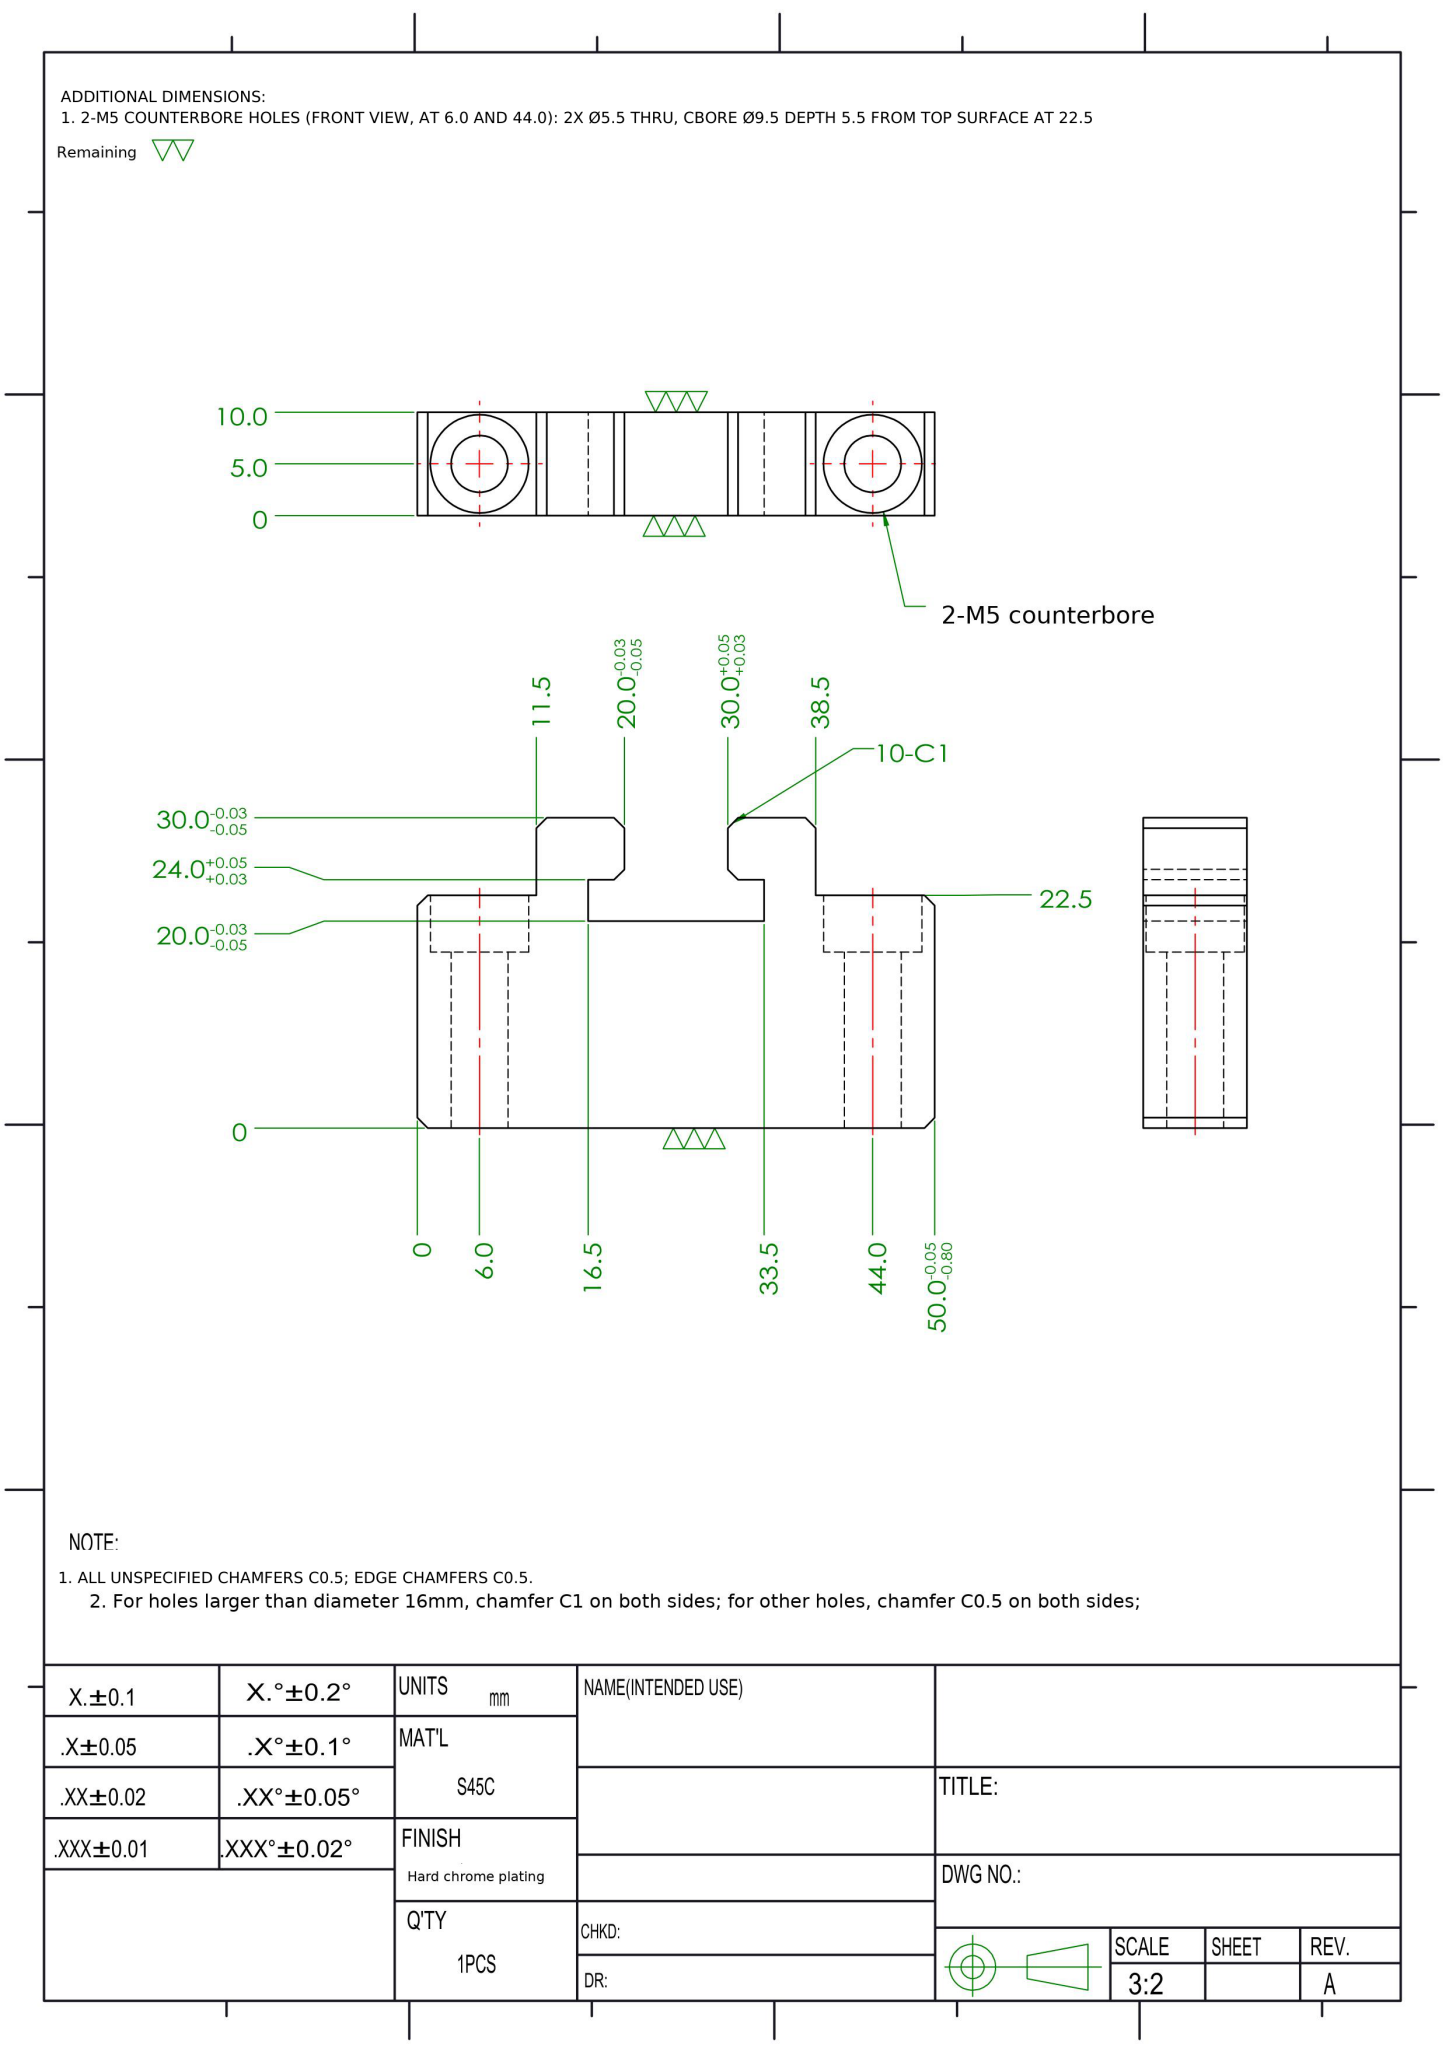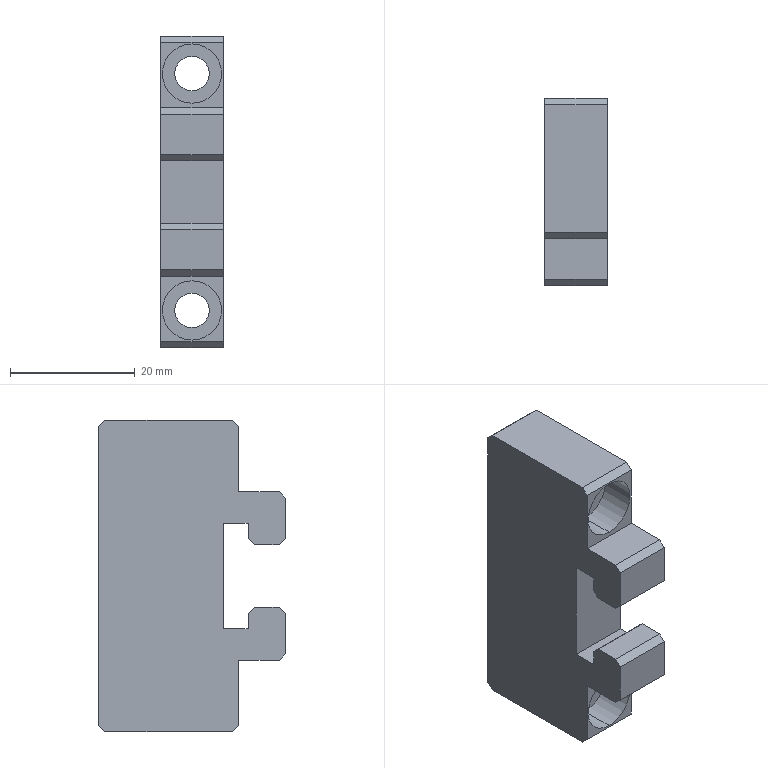Part | NX | mm | 1 solid | 38 faces | box 10 x 30 x 50 mm | volume 10358 mm3 | plane 30 | cylinder 8 | commonest cylinder face diameters 9.5 x4 5.5 x4